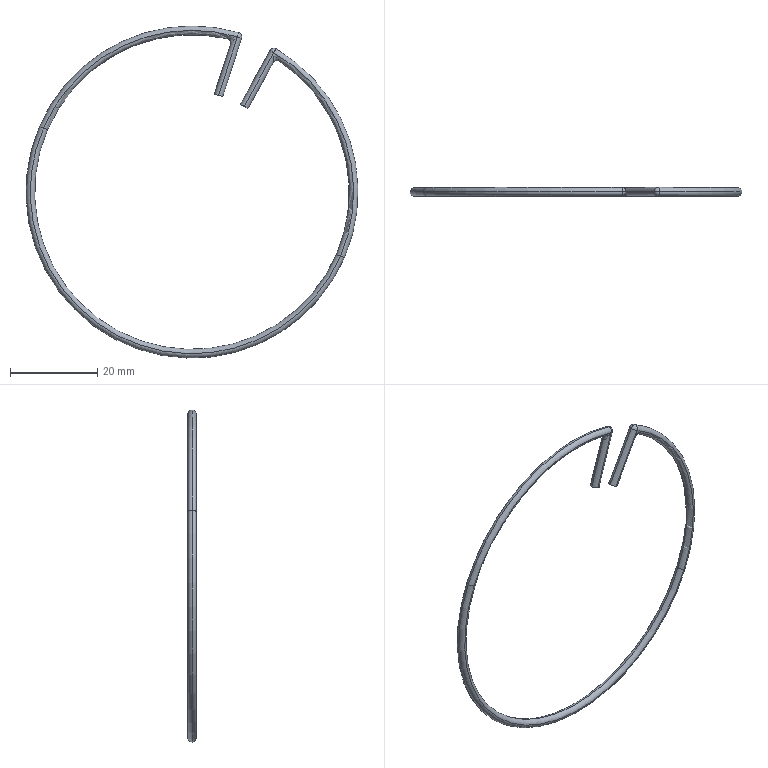Component | SolidWorks | Cache Festo AD85-2_Circlips-1 | 1 solid | 30 faces | box 76 x 2 x 76 mm | volume 790 mm3 | torus 12 | cylinder 8 | spline 4 | sphere 4 | plane 2 | commonest cylinder face diameters 2 x8